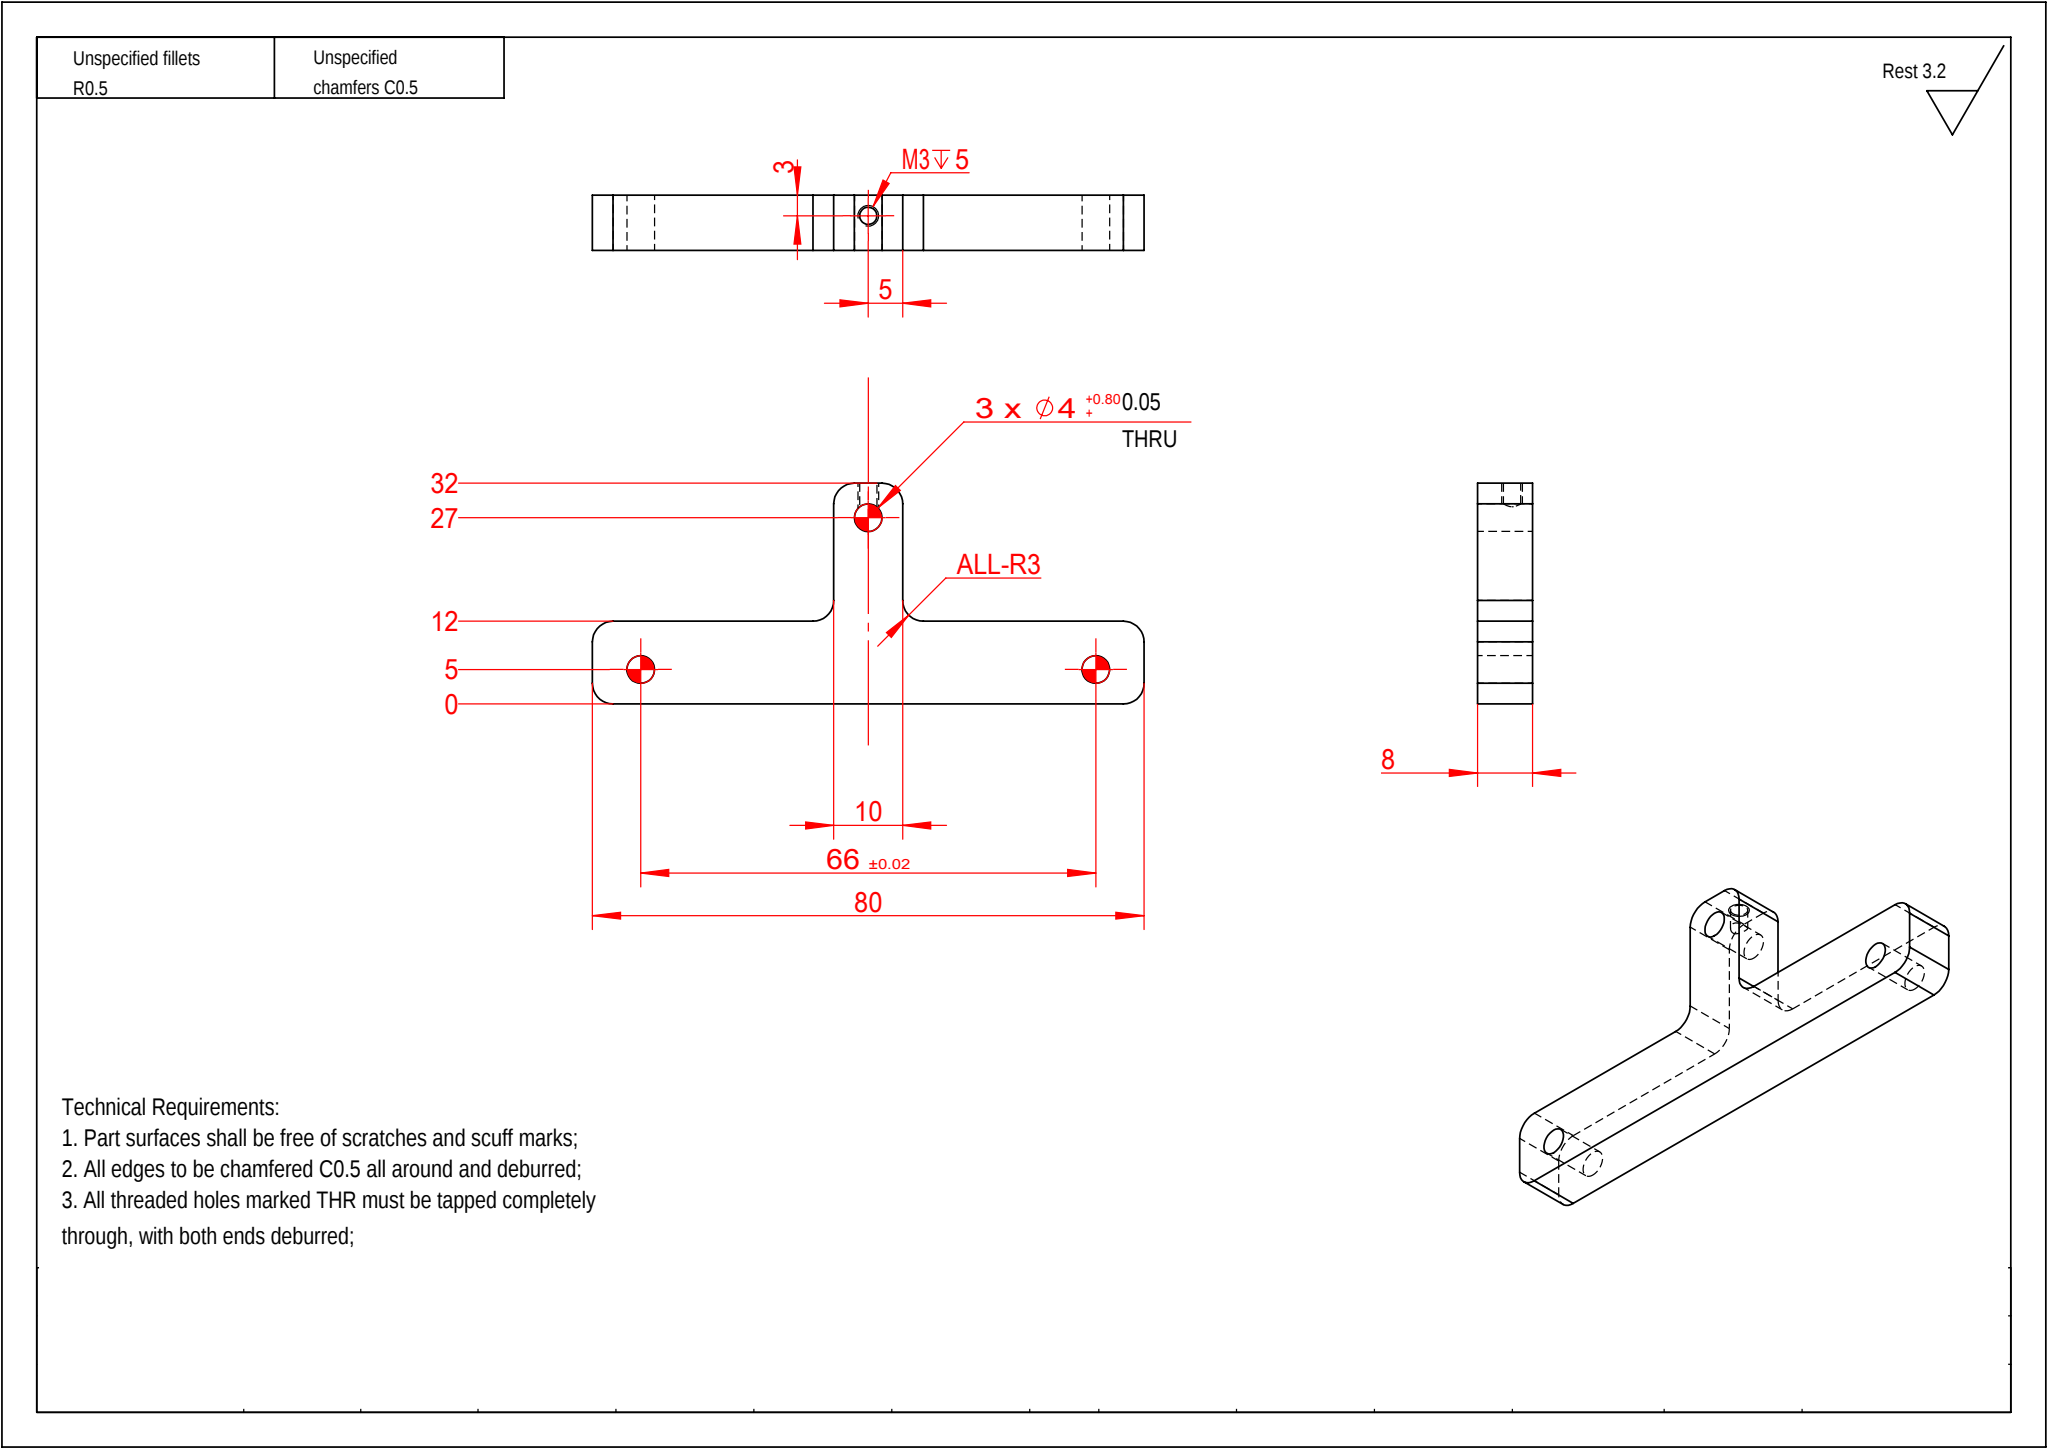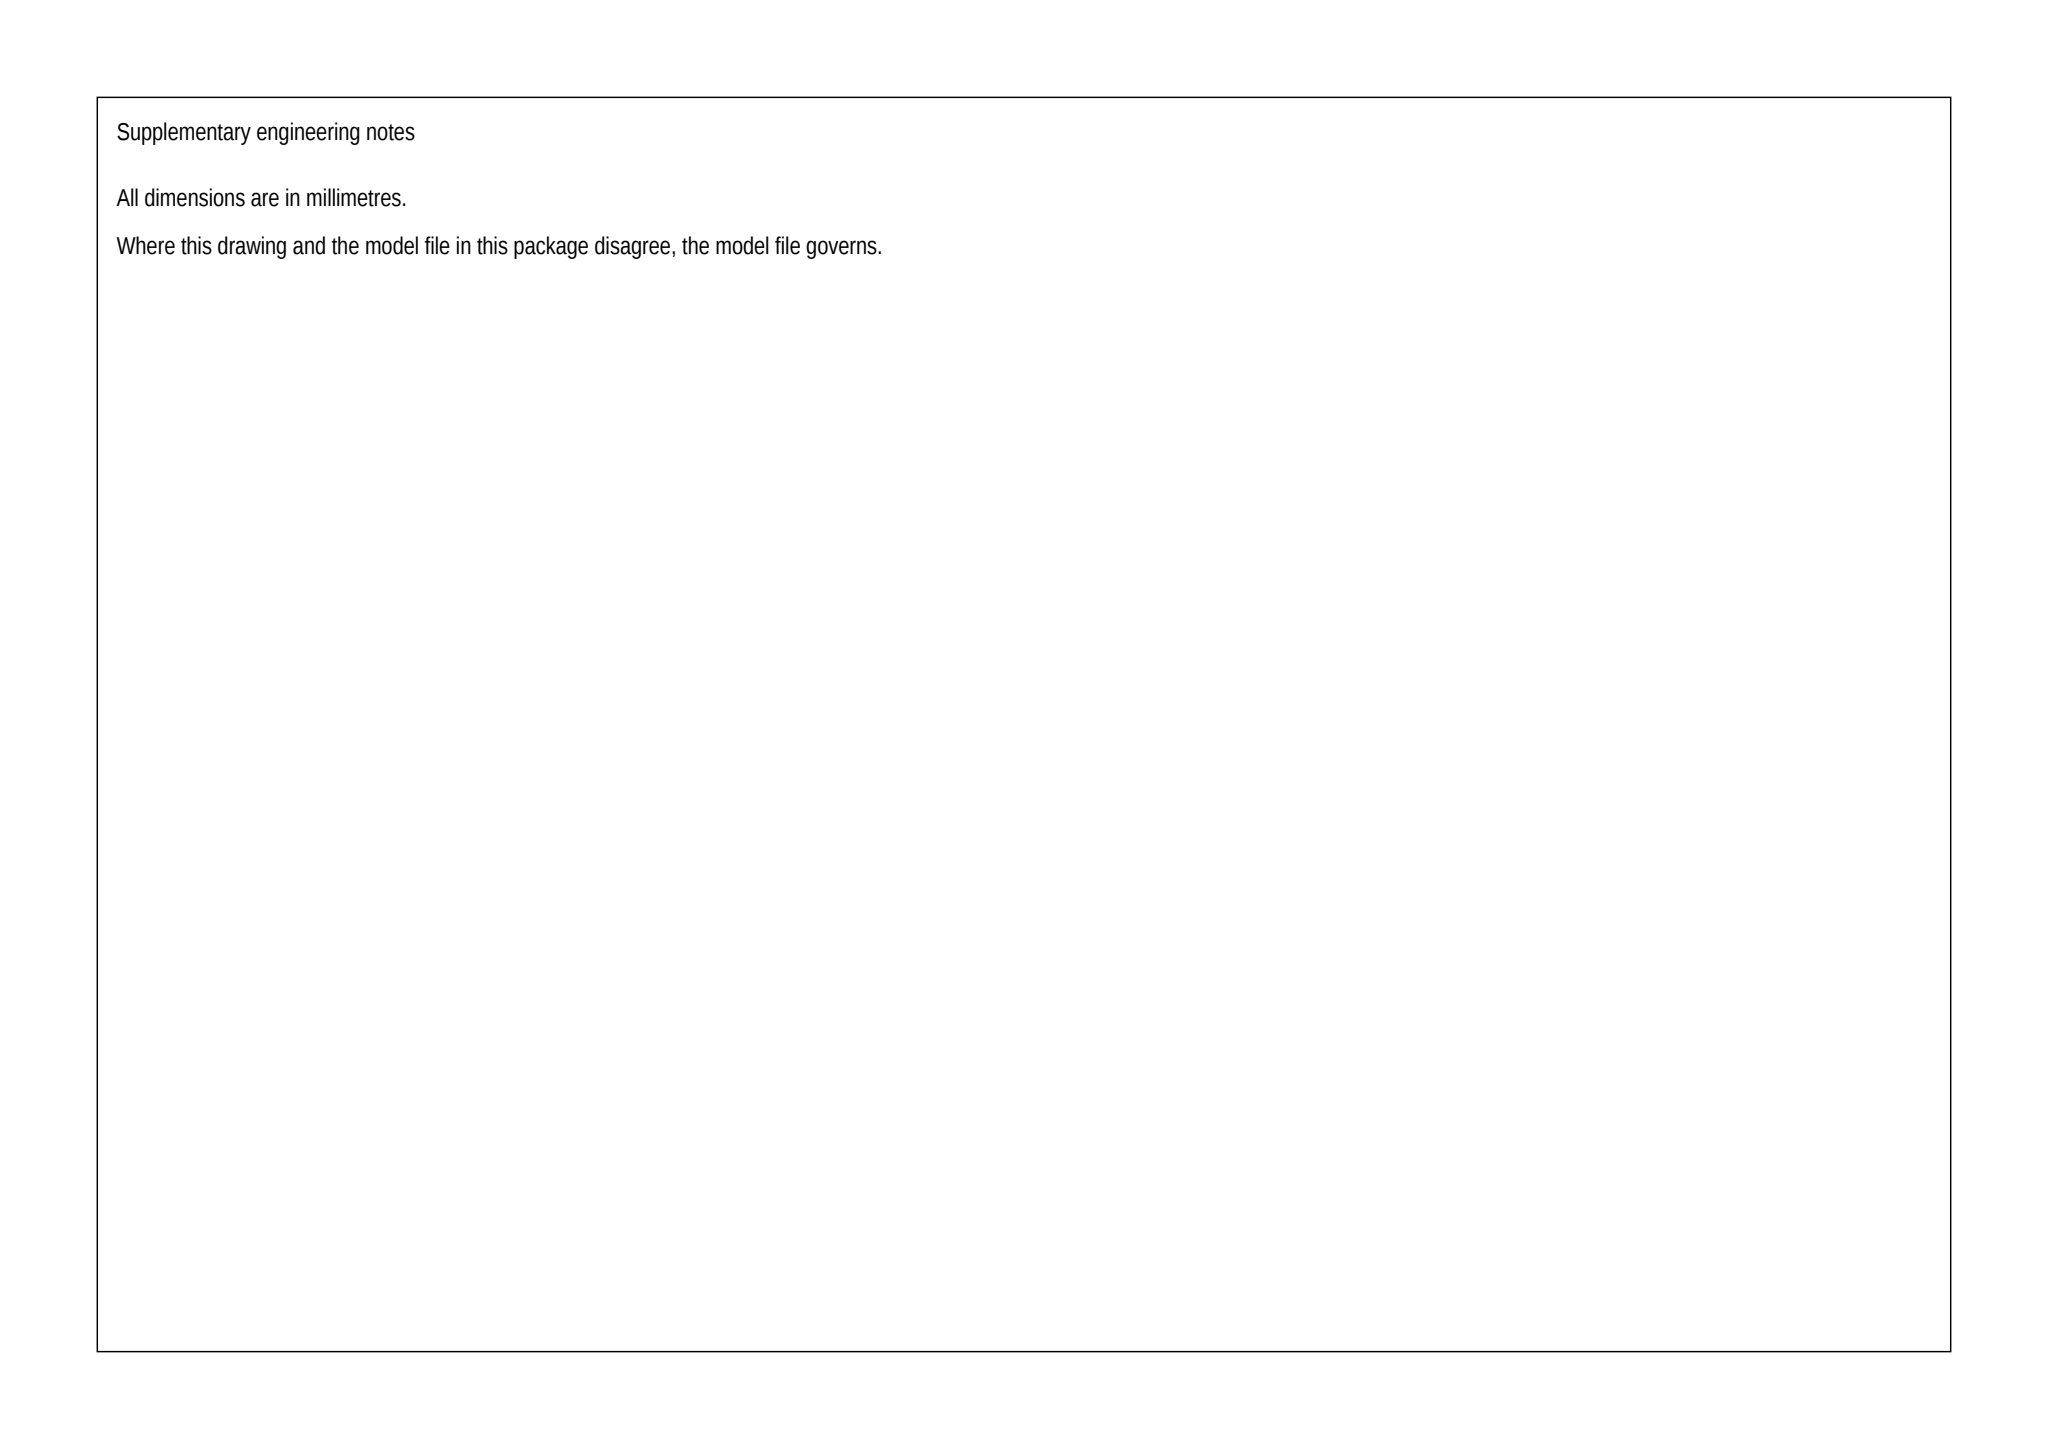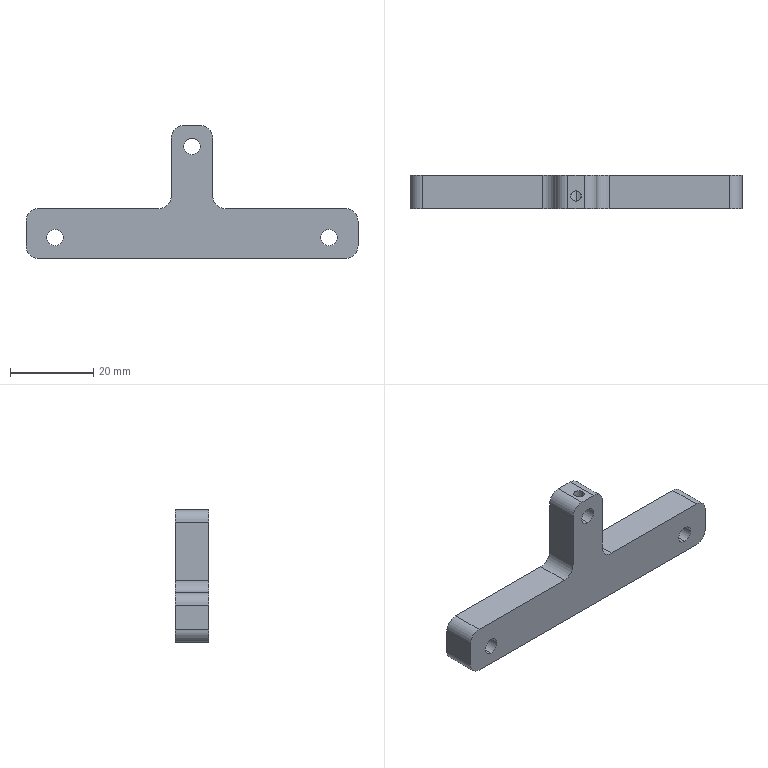Part | SolidWorks | mm | 1 solid | 26 faces | box 80 x 8 x 32 mm | volume 8901 mm3 | cylinder 16 | plane 10 | commonest cylinder face diameters 6 x8 4 x6 2.5 x2
Drawing notes:
2. ALL EDGES/CORNERS C0.5 ALL AROUND | from the solid: No fillet radii in STEP; all sharp edges per default chamfer C0.5 note
3. ALL THR TAPPED HOLES TAPPED FULL THRU, DEBURR BOTH ENDS | from the solid: Thru features span full 8 thk (cyl len 8 along Y, bbox Y=8)
3 x Ø4 +0.08/+0.05 THRU | from the solid: Three Ø4 Y-axis cyls len 8 = full 8 thk at (7,5), (40,27), (73,5)
build123d program:
from build123d import *

# Parameters (mm, degrees)
SKETCH1_W              = 80
SKETCH1_H              = 12
BOSS_EXTRUDE1_DEPTH    = 8
SKETCH2_W              = 10
SKETCH2_H              = 20
BOSS_EXTRUDE2_DEPTH    = 8
SKETCH3_R              = 2
CUT_EXTRUDE1_DEPTH     = 49.374
SKETCH4_R              = 2
CUT_EXTRUDE2_DEPTH     = 49.374
FILLET1_R              = 3
M3_TAPPED_HOLE1_REACH  = 53.846
M3_TAPPED_HOLE1_BORE_R = 1.25


with BuildPart() as part:
    # Sketch1 → Boss-Extrude1 (new body)
    with BuildSketch(Plane(origin=(0, 0, 0), x_dir=(1, 0, 0), z_dir=(0, 1, 0))):
        Rectangle(SKETCH1_W, SKETCH1_H)
    extrude(amount=BOSS_EXTRUDE1_DEPTH)

    # Sketch2 → Boss-Extrude2 (add)
    with BuildSketch(Plane(origin=(0, 8, 0), x_dir=(1, 0, 0), z_dir=(0, 1, 0))):
        with Locations((0, -16)):
            Rectangle(SKETCH2_W, SKETCH2_H)
    extrude(amount=-BOSS_EXTRUDE2_DEPTH)

    # Sketch3 → Cut-Extrude1 (cut, through all)
    with BuildSketch(Plane.XZ):
        with Locations(Location((-33, -1, 0), (0, 0, 270))):
            Circle(SKETCH3_R)
    cut_extrude1 = extrude(amount=-CUT_EXTRUDE1_DEPTH, mode=Mode.SUBTRACT)

    # Mirror1: Cut-Extrude1 across plane
    add(cut_extrude1.mirror(Plane(origin=(0, 0, 0), x_dir=(0, 0, 1), z_dir=(1, 0, 0))), mode=Mode.SUBTRACT)

    # Sketch4 → Cut-Extrude2 (cut, through all)
    with BuildSketch(Plane.XZ):
        with Locations(Location((0, 21, 0), (0, 0, 270))):
            Circle(SKETCH4_R)
    extrude(amount=-CUT_EXTRUDE2_DEPTH, mode=Mode.SUBTRACT)

    # Fillet1
    fillet1_edges = [part.edges().sort_by_distance(p)[0] for p in [
        (5, 4, 6),
        (5, 4, 26),
        (-5, 4, 26),
        (-5, 4, 6),
        (40, 4, 6),
        (-40, 4, 6),
        (-40, 4, -6),
        (40, 4, -6),
    ]]
    fillet(fillet1_edges, radius=FILLET1_R)

    # M3 Tapped Hole1 bore → M3 Tapped Hole1 (cut, up to next)
    with BuildSketch(Plane.XY.offset(26), mode=Mode.PRIVATE) as m3_tapped_hole1_sk1:
        with Locations((0, 3)):
            Circle(M3_TAPPED_HOLE1_BORE_R)
    m3_tapped_hole1_tool1 = extrude(m3_tapped_hole1_sk1.sketch, amount=-M3_TAPPED_HOLE1_REACH, mode=Mode.PRIVATE) & part.part
    add(m3_tapped_hole1_tool1.solids().sort_by_distance((0, 3, 26))[0], mode=Mode.SUBTRACT)


solid = part.part